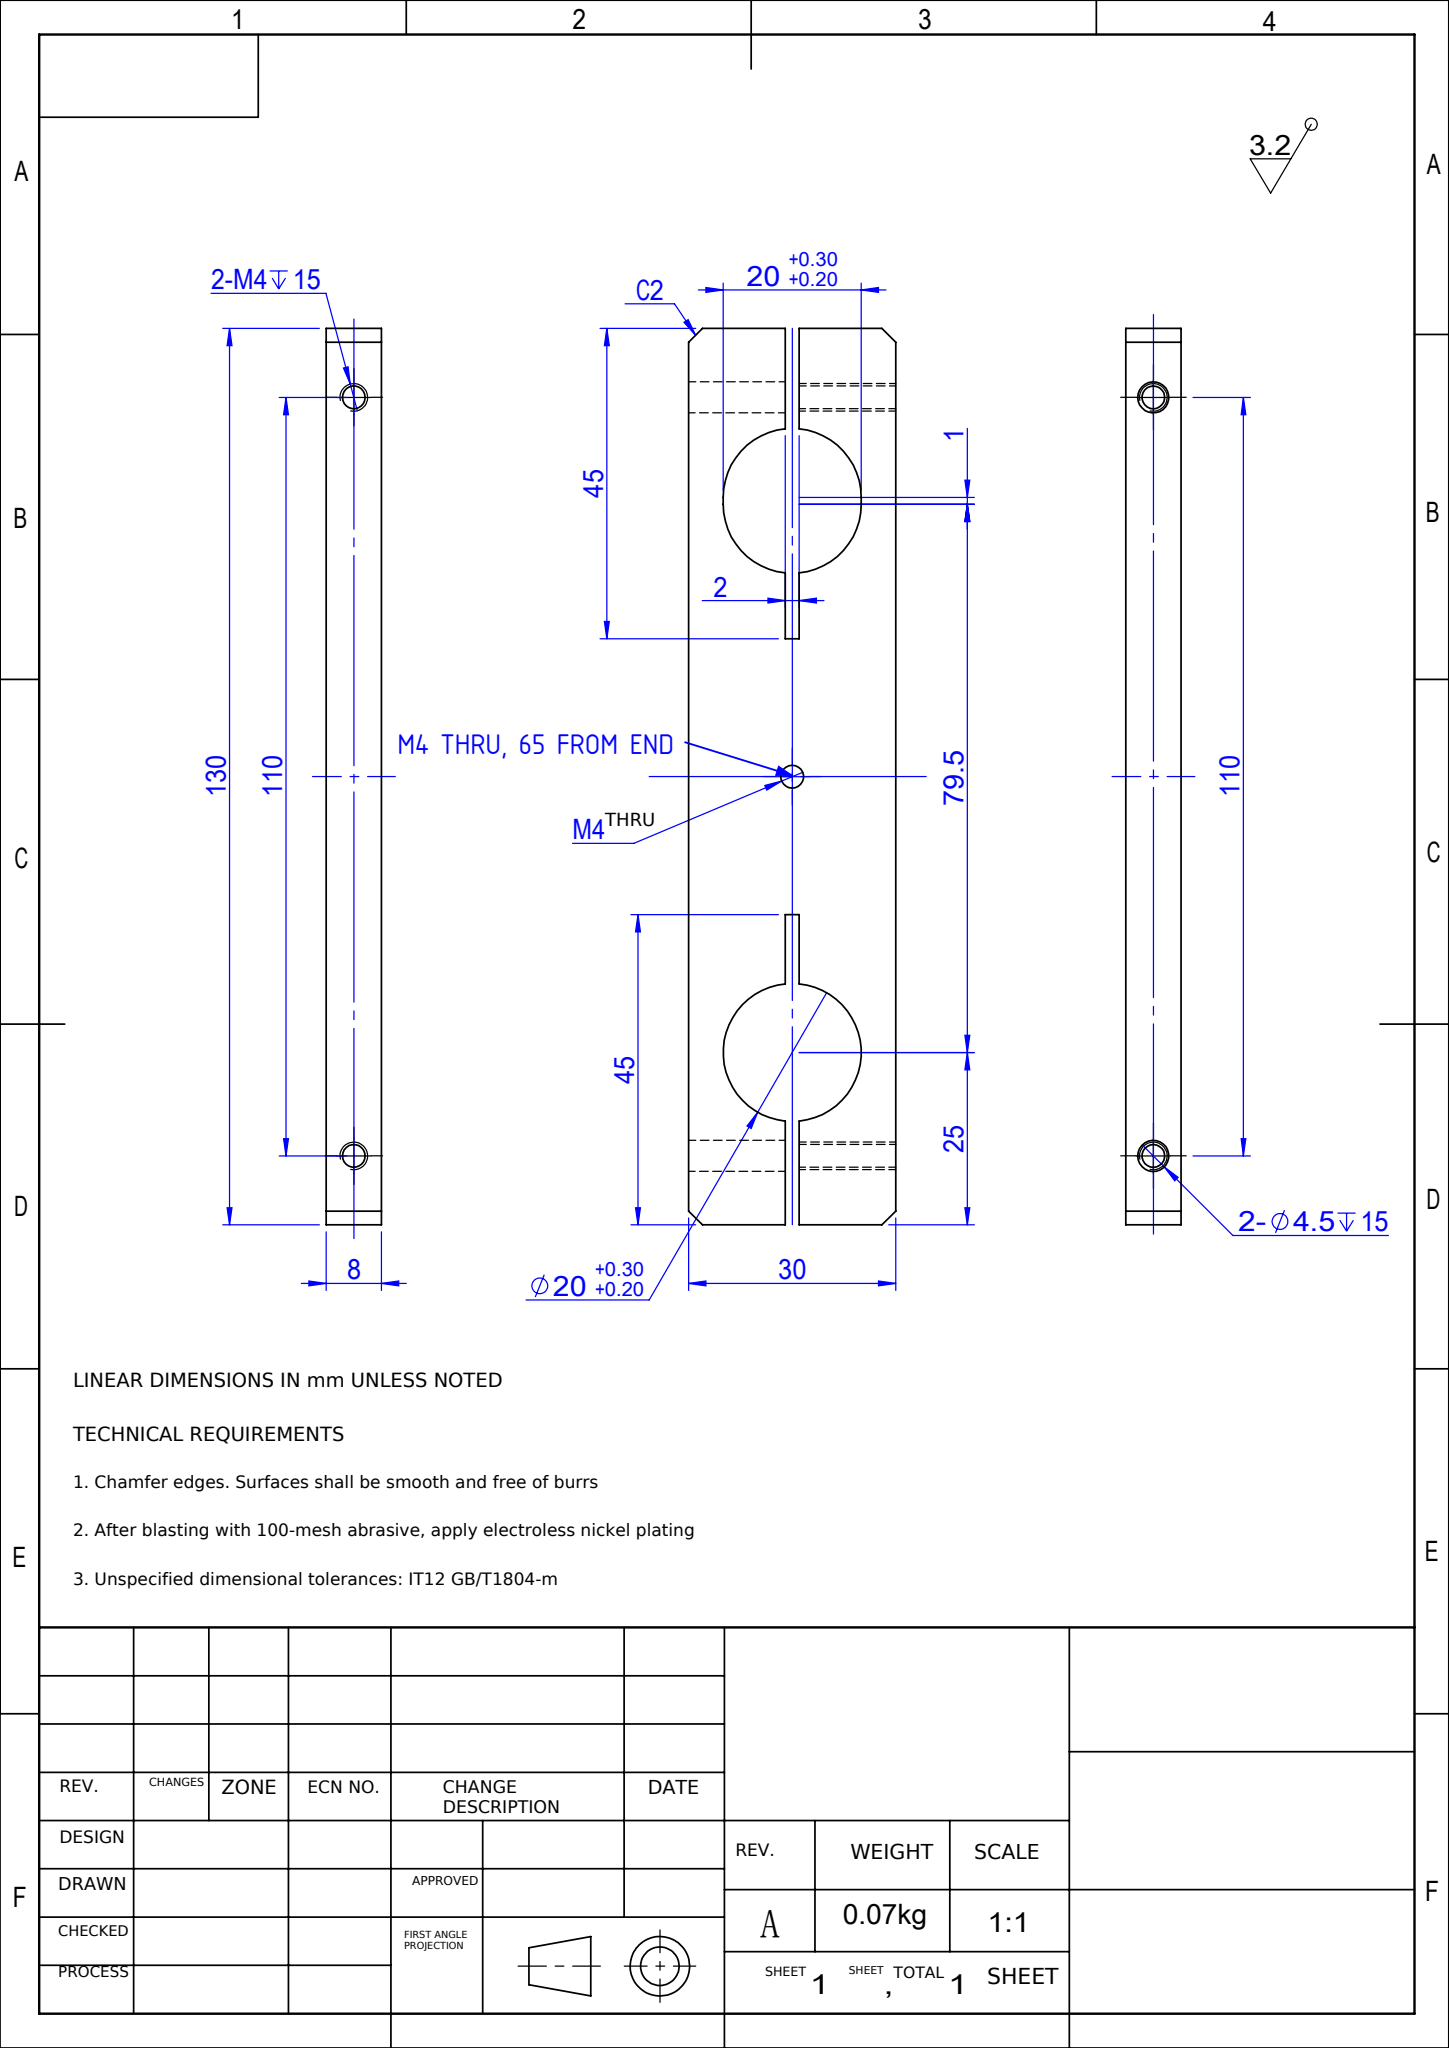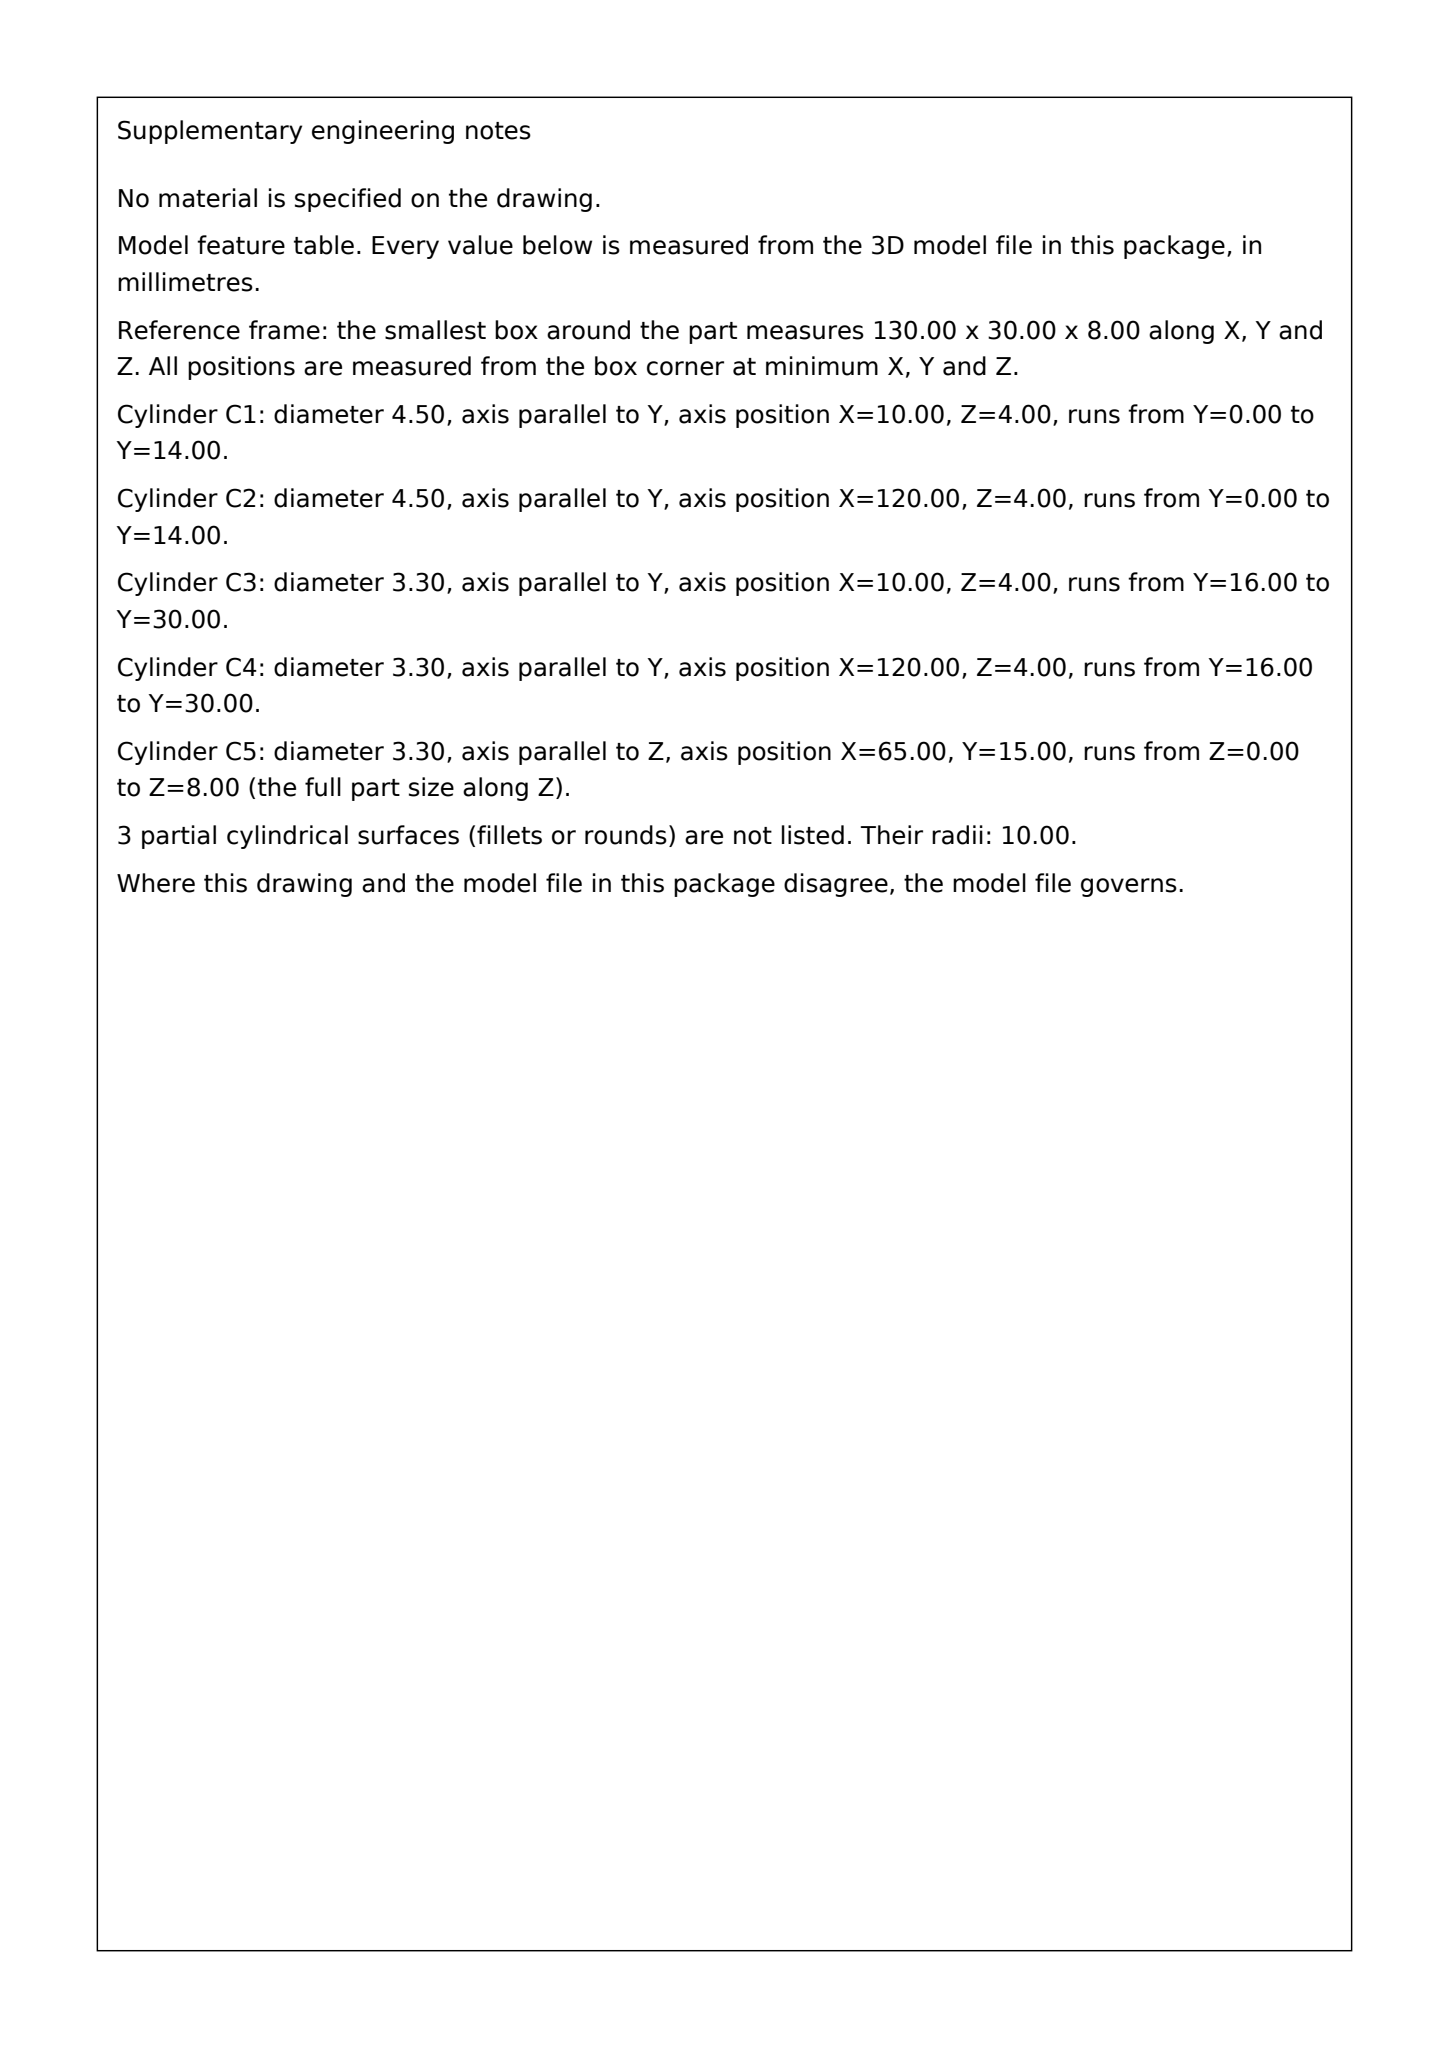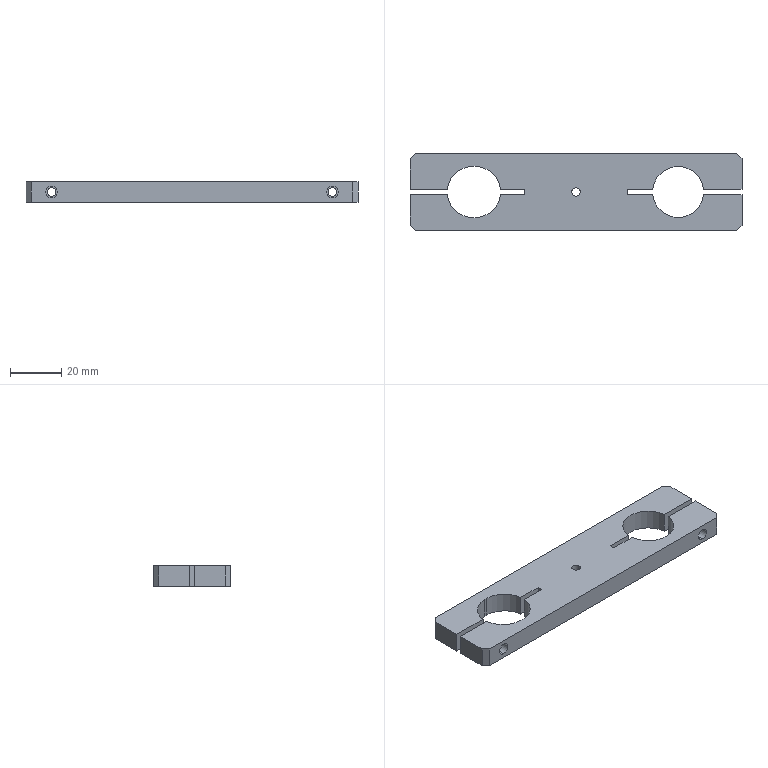Part | SolidWorks | mm | 1 solid | 40 faces | box 130 x 30 x 8 mm | volume 24411 mm3 | plane 24 | cylinder 16 | commonest cylinder face diameters 3.3 x6 20 x6 4.5 x4
Drawing notes:
M4 THRU (CENTER HOLE, 65 FROM END) | from the solid: hole/bore dia 3.3, axis z at (65,15), from z=0 to z=8 (full 8 thk)
build123d program:
from build123d import *

# Parameters (mm, degrees)
SKETCH1_W                  = 130
SKETCH1_H                  = 30
BOSS_EXTRUDE1_DEPTH        = 8
F_20_0_20_DIAMETER_HOLE1_D = 20
CHAMFER1_SIZE              = 2
CUT_EXTRUDE2_DEPTH         = 68.186
SKETCH6_W                  = 45
SKETCH6_H                  = 2
CUT_EXTRUDE1_DEPTH         = 68.186
M4_TAPPED_HOLE2_D          = 3.3
M4_TAPPED_HOLE2_DEPTH      = 14
M4_CLEARANCE_HOLE1_D       = 4.5
M4_CLEARANCE_HOLE1_DEPTH   = 14
M4_TAPPED_HOLE3_D          = 3.3


with BuildPart() as part:
    # Sketch1 → Boss-Extrude1 (new body)
    with BuildSketch(Plane.XY):
        Rectangle(SKETCH1_W, SKETCH1_H)
    extrude(amount=BOSS_EXTRUDE1_DEPTH)

    # 20.0 _20_ Diameter Hole1 (through all)
    with Locations(Plane.XY.offset(8)):
        with Locations((40, 0)):
            Hole(F_20_0_20_DIAMETER_HOLE1_D / 2)

    # Chamfer1
    chamfer1_edges = [part.edges().sort_by_distance(p)[0] for p in [
        (-65, 15, 4),
        (65, 15, 4),
        (65, -15, 4),
        (-65, -15, 4),
    ]]
    chamfer(chamfer1_edges, length=CHAMFER1_SIZE)

    # Sketch14 → Cut-Extrude2 (cut, through all)
    with BuildSketch(Plane(origin=(0, 0, 0), x_dir=(-1, 0, 0), z_dir=(0, 0, -1))):
        with BuildLine():
            Line((39.5, 10), (40.5, 10))
            ThreePointArc((40.5, 10), (50.5, 0), (40.5, -10))
            Line((40.5, -10), (39.5, -10))
            ThreePointArc((39.5, -10), (29.5, 0), (39.5, 10))
        make_face()
    extrude(amount=-CUT_EXTRUDE2_DEPTH, mode=Mode.SUBTRACT)

    # Sketch6 → Cut-Extrude1 (cut, through all)
    with BuildSketch(Plane.XY.offset(8)):
        with Locations((42.5, 0)):
            Rectangle(SKETCH6_W, SKETCH6_H)
        with Locations((-42.5, 0)):
            Rectangle(SKETCH6_W, SKETCH6_H)
    extrude(amount=-CUT_EXTRUDE1_DEPTH, mode=Mode.SUBTRACT)

    # M4 Tapped Hole2
    with Locations(Plane(origin=(0, 15, 0), x_dir=(-1, 0, 0), z_dir=(0, 1, 0))):
        with Locations((55, 4), (-55, 4)):
            Hole(M4_TAPPED_HOLE2_D / 2, depth=M4_TAPPED_HOLE2_DEPTH)

    # M4 Clearance Hole1
    with Locations(Plane.XZ.offset(15)):
        with Locations((-55, 4), (55, 4)):
            Hole(M4_CLEARANCE_HOLE1_D / 2, depth=M4_CLEARANCE_HOLE1_DEPTH)

    # M4 Tapped Hole3 (through all)
    with Locations(Plane.XY.offset(8)):
        with Locations((0, 0)):
            Hole(M4_TAPPED_HOLE3_D / 2)


solid = part.part